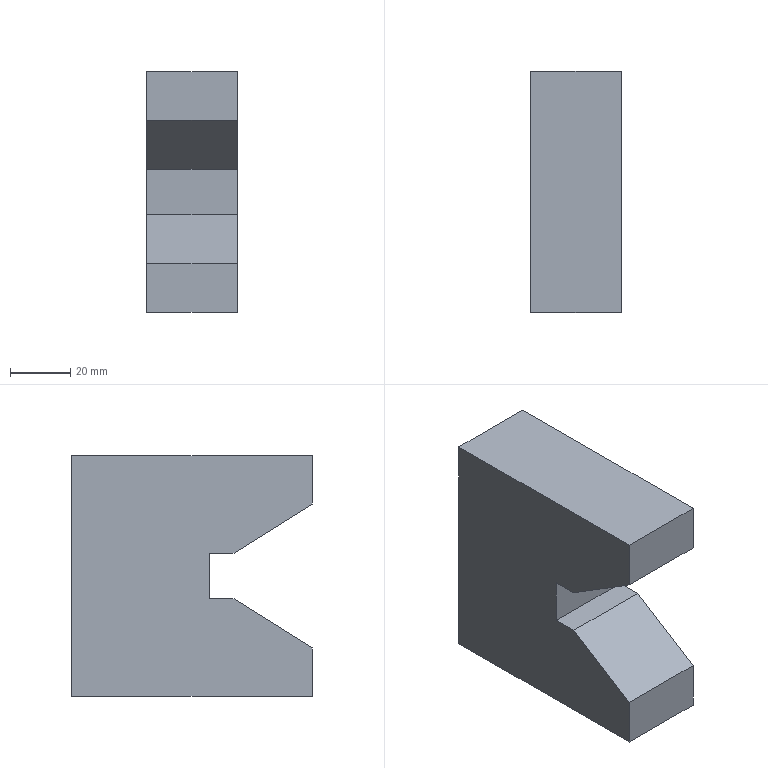Component | NX | MOVABLE_V_BLOCK | 1 solid | 14 faces | box 30 x 80 x 80 mm | volume 162754 mm3 | plane 13 | cylinder 1 | commonest cylinder face diameters 15 x1
STEP:
#1=CARTESIAN_POINT('',(0.,0.,0.));
#2=DIRECTION('',(0.,0.,1.));
#3=DIRECTION('',(1.,0.,0.));
#4=AXIS2_PLACEMENT_3D('',#1,#2,#3);
#5=CARTESIAN_POINT('',(39.511,118.604,6.098));
#6=VERTEX_POINT('',#5);
#7=CARTESIAN_POINT('',(39.511,144.658,22.378));
#8=VERTEX_POINT('',#7);
#9=CARTESIAN_POINT('',(39.511,118.604,6.098));
#10=DIRECTION('',(0.,0.848,0.5299));
#11=VECTOR('',#10,1.);
#12=LINE('',#9,#11);
#13=CARTESIAN_POINT('',(39.511,118.604,-10.));
#14=DIRECTION('',(-1.,0.,0.));
#15=DIRECTION('',(0.,-1.,0.));
#16=AXIS2_PLACEMENT_3D('',#13,#14,#15);
#17=PLANE('',#16);
#18=CARTESIAN_POINT('',(0.,16.098));
#19=DIRECTION('',(-0.848,0.5299));
#20=VECTOR('',#19,1.);
#21=LINE('',#18,#20);
#22=(GEOMETRIC_REPRESENTATION_CONTEXT(2)PARAMETRIC_REPRESENTATION_CONTEXT()REPRESENTATION_CONTEXT('',''));
#23=DEFINITIONAL_REPRESENTATION('',(#21),#22);
#24=PCURVE('',#17,#23);
#25=CARTESIAN_POINT('',(-280.489,118.604,6.098));
#26=DIRECTION('',(0.,0.5299,-0.848));
#27=DIRECTION('',(0.,-0.848,-0.5299));
#28=AXIS2_PLACEMENT_3D('',#25,#26,#27);
#29=PLANE('',#28);
#30=CARTESIAN_POINT('',(0.,-320.));
#31=DIRECTION('',(-1.,0.));
#32=VECTOR('',#31,1.);
#33=LINE('',#30,#32);
#34=(GEOMETRIC_REPRESENTATION_CONTEXT(2)PARAMETRIC_REPRESENTATION_CONTEXT()REPRESENTATION_CONTEXT('',''));
#35=DEFINITIONAL_REPRESENTATION('',(#33),#34);
#36=PCURVE('',#29,#35);
#37=SURFACE_CURVE('',#12,(#24,#36),.PCURVE_S1.);
#38=EDGE_CURVE('',#6,#8,#37,.T.);
#39=ORIENTED_EDGE('',*,*,#38,.F.);
#40=CARTESIAN_POINT('',(39.511,118.604,-10.));
#41=VERTEX_POINT('',#40);
#42=CARTESIAN_POINT('',(39.511,118.604,-10.));
#43=DIRECTION('',(0.,0.,1.));
#44=VECTOR('',#43,1.);
#45=LINE('',#42,#44);
#46=CARTESIAN_POINT('',(0.,0.));
#47=DIRECTION('',(0.,1.));
#48=VECTOR('',#47,1.);
#49=LINE('',#46,#48);
#50=(GEOMETRIC_REPRESENTATION_CONTEXT(2)PARAMETRIC_REPRESENTATION_CONTEXT()REPRESENTATION_CONTEXT('',''));
#51=DEFINITIONAL_REPRESENTATION('',(#49),#50);
#52=PCURVE('',#17,#51);
#53=CARTESIAN_POINT('',(39.511,118.604,-10.));
#54=DIRECTION('',(0.,-1.,0.));
#55=DIRECTION('',(0.,0.,1.));
#56=AXIS2_PLACEMENT_3D('',#53,#54,#55);
#57=PLANE('',#56);
#58=CARTESIAN_POINT('',(0.,0.));
#59=DIRECTION('',(1.,0.));
#60=VECTOR('',#59,1.);
#61=LINE('',#58,#60);
#62=(GEOMETRIC_REPRESENTATION_CONTEXT(2)PARAMETRIC_REPRESENTATION_CONTEXT()REPRESENTATION_CONTEXT('',''));
#63=DEFINITIONAL_REPRESENTATION('',(#61),#62);
#64=PCURVE('',#57,#63);
#65=SURFACE_CURVE('',#45,(#52,#64),.PCURVE_S1.);
#66=EDGE_CURVE('',#41,#6,#65,.T.);
#67=ORIENTED_EDGE('',*,*,#66,.F.);
#68=CARTESIAN_POINT('',(39.511,198.604,-10.));
#69=VERTEX_POINT('',#68);
#70=CARTESIAN_POINT('',(39.511,118.604,-10.));
#71=DIRECTION('',(0.,1.,0.));
#72=VECTOR('',#71,1.);
#73=LINE('',#70,#72);
#74=CARTESIAN_POINT('',(0.,0.));
#75=DIRECTION('',(-1.,0.));
#76=VECTOR('',#75,1.);
#77=LINE('',#74,#76);
#78=(GEOMETRIC_REPRESENTATION_CONTEXT(2)PARAMETRIC_REPRESENTATION_CONTEXT()REPRESENTATION_CONTEXT('',''));
#79=DEFINITIONAL_REPRESENTATION('',(#77),#78);
#80=PCURVE('',#17,#79);
#81=CARTESIAN_POINT('',(9.511,118.604,-10.));
#82=DIRECTION('',(0.,0.,1.));
#83=DIRECTION('',(-1.,0.,0.));
#84=AXIS2_PLACEMENT_3D('',#81,#82,#83);
#85=PLANE('',#84);
#86=CARTESIAN_POINT('',(-30.,0.));
#87=DIRECTION('',(0.,-1.));
#88=VECTOR('',#87,1.);
#89=LINE('',#86,#88);
#90=(GEOMETRIC_REPRESENTATION_CONTEXT(2)PARAMETRIC_REPRESENTATION_CONTEXT()REPRESENTATION_CONTEXT('',''));
#91=DEFINITIONAL_REPRESENTATION('',(#89),#90);
#92=PCURVE('',#85,#91);
#93=SURFACE_CURVE('',#73,(#80,#92),.PCURVE_S1.);
#94=EDGE_CURVE('',#41,#69,#93,.T.);
#95=ORIENTED_EDGE('',*,*,#94,.T.);
#96=CARTESIAN_POINT('',(39.511,198.604,70.));
#97=VERTEX_POINT('',#96);
#98=CARTESIAN_POINT('',(39.511,198.604,-10.));
#99=DIRECTION('',(0.,0.,1.));
#100=VECTOR('',#99,1.);
#101=LINE('',#98,#100);
#102=CARTESIAN_POINT('',(-80.,0.));
#103=DIRECTION('',(0.,1.));
#104=VECTOR('',#103,1.);
#105=LINE('',#102,#104);
#106=(GEOMETRIC_REPRESENTATION_CONTEXT(2)PARAMETRIC_REPRESENTATION_CONTEXT()REPRESENTATION_CONTEXT('',''));
#107=DEFINITIONAL_REPRESENTATION('',(#105),#106);
#108=PCURVE('',#17,#107);
#109=CARTESIAN_POINT('',(39.511,198.604,-10.));
#110=DIRECTION('',(0.,-1.,0.));
#111=DIRECTION('',(0.,0.,1.));
#112=AXIS2_PLACEMENT_3D('',#109,#110,#111);
#113=PLANE('',#112);
#114=CARTESIAN_POINT('',(0.,0.));
#115=DIRECTION('',(1.,0.));
#116=VECTOR('',#115,1.);
#117=LINE('',#114,#116);
#118=(GEOMETRIC_REPRESENTATION_CONTEXT(2)PARAMETRIC_REPRESENTATION_CONTEXT()REPRESENTATION_CONTEXT('',''));
#119=DEFINITIONAL_REPRESENTATION('',(#117),#118);
#120=PCURVE('',#113,#119);
#121=SURFACE_CURVE('',#101,(#108,#120),.PCURVE_S1.);
#122=EDGE_CURVE('',#69,#97,#121,.T.);
#123=ORIENTED_EDGE('',*,*,#122,.T.);
#124=CARTESIAN_POINT('',(39.511,118.604,70.));
#125=VERTEX_POINT('',#124);
#126=CARTESIAN_POINT('',(39.511,118.604,70.));
#127=DIRECTION('',(0.,1.,0.));
#128=VECTOR('',#127,1.);
#129=LINE('',#126,#128);
#130=CARTESIAN_POINT('',(0.,80.));
#131=DIRECTION('',(-1.,0.));
#132=VECTOR('',#131,1.);
#133=LINE('',#130,#132);
#134=(GEOMETRIC_REPRESENTATION_CONTEXT(2)PARAMETRIC_REPRESENTATION_CONTEXT()REPRESENTATION_CONTEXT('',''));
#135=DEFINITIONAL_REPRESENTATION('',(#133),#134);
#136=PCURVE('',#17,#135);
#137=CARTESIAN_POINT('',(39.511,118.604,70.));
#138=DIRECTION('',(0.,0.,-1.));
#139=DIRECTION('',(0.,-1.,0.));
#140=AXIS2_PLACEMENT_3D('',#137,#138,#139);
#141=PLANE('',#140);
#142=CARTESIAN_POINT('',(0.,0.));
#143=DIRECTION('',(-1.,0.));
#144=VECTOR('',#143,1.);
#145=LINE('',#142,#144);
#146=(GEOMETRIC_REPRESENTATION_CONTEXT(2)PARAMETRIC_REPRESENTATION_CONTEXT()REPRESENTATION_CONTEXT('',''));
#147=DEFINITIONAL_REPRESENTATION('',(#145),#146);
#148=PCURVE('',#141,#147);
#149=SURFACE_CURVE('',#129,(#136,#148),.PCURVE_S1.);
#150=EDGE_CURVE('',#125,#97,#149,.T.);
#151=ORIENTED_EDGE('',*,*,#150,.F.);
#152=CARTESIAN_POINT('',(39.511,118.604,53.902));
#153=VERTEX_POINT('',#152);
#154=CARTESIAN_POINT('',(39.511,118.604,-10.));
#155=DIRECTION('',(0.,0.,1.));
#156=VECTOR('',#155,1.);
#157=LINE('',#154,#156);
#158=CARTESIAN_POINT('',(0.,0.));
#159=DIRECTION('',(0.,1.));
#160=VECTOR('',#159,1.);
#161=LINE('',#158,#160);
#162=(GEOMETRIC_REPRESENTATION_CONTEXT(2)PARAMETRIC_REPRESENTATION_CONTEXT()REPRESENTATION_CONTEXT('',''));
#163=DEFINITIONAL_REPRESENTATION('',(#161),#162);
#164=PCURVE('',#17,#163);
#165=CARTESIAN_POINT('',(39.511,118.604,-10.));
#166=DIRECTION('',(0.,-1.,0.));
#167=DIRECTION('',(0.,0.,1.));
#168=AXIS2_PLACEMENT_3D('',#165,#166,#167);
#169=PLANE('',#168);
#170=CARTESIAN_POINT('',(0.,0.));
#171=DIRECTION('',(1.,0.));
#172=VECTOR('',#171,1.);
#173=LINE('',#170,#172);
#174=(GEOMETRIC_REPRESENTATION_CONTEXT(2)PARAMETRIC_REPRESENTATION_CONTEXT()REPRESENTATION_CONTEXT('',''));
#175=DEFINITIONAL_REPRESENTATION('',(#173),#174);
#176=PCURVE('',#169,#175);
#177=SURFACE_CURVE('',#157,(#164,#176),.PCURVE_S1.);
#178=EDGE_CURVE('',#153,#125,#177,.T.);
#179=ORIENTED_EDGE('',*,*,#178,.F.);
#180=CARTESIAN_POINT('',(39.511,144.658,37.622));
#181=VERTEX_POINT('',#180);
#182=CARTESIAN_POINT('',(39.511,144.658,37.622));
#183=DIRECTION('',(0.,-0.848,0.5299));
#184=VECTOR('',#183,1.);
#185=LINE('',#182,#184);
#186=CARTESIAN_POINT('',(-26.054,47.622));
#187=DIRECTION('',(0.848,0.5299));
#188=VECTOR('',#187,1.);
#189=LINE('',#186,#188);
#190=(GEOMETRIC_REPRESENTATION_CONTEXT(2)PARAMETRIC_REPRESENTATION_CONTEXT()REPRESENTATION_CONTEXT('',''));
#191=DEFINITIONAL_REPRESENTATION('',(#189),#190);
#192=PCURVE('',#17,#191);
#193=CARTESIAN_POINT('',(-280.489,144.658,37.622));
#194=DIRECTION('',(0.,0.5299,0.848));
#195=DIRECTION('',(0.,0.848,-0.5299));
#196=AXIS2_PLACEMENT_3D('',#193,#194,#195);
#197=PLANE('',#196);
#198=CARTESIAN_POINT('',(0.,-320.));
#199=DIRECTION('',(-1.,0.));
#200=VECTOR('',#199,1.);
#201=LINE('',#198,#200);
#202=(GEOMETRIC_REPRESENTATION_CONTEXT(2)PARAMETRIC_REPRESENTATION_CONTEXT()REPRESENTATION_CONTEXT('',''));
#203=DEFINITIONAL_REPRESENTATION('',(#201),#202);
#204=PCURVE('',#197,#203);
#205=SURFACE_CURVE('',#185,(#192,#204),.PCURVE_S1.);
#206=EDGE_CURVE('',#181,#153,#205,.T.);
#207=ORIENTED_EDGE('',*,*,#206,.F.);
#208=CARTESIAN_POINT('',(39.511,152.798,37.622));
#209=VERTEX_POINT('',#208);
#210=CARTESIAN_POINT('',(39.511,152.798,37.622));
#211=DIRECTION('',(0.,-1.,0.));
#212=VECTOR('',#211,1.);
#213=LINE('',#210,#212);
#214=CARTESIAN_POINT('',(-34.194,47.622));
#215=DIRECTION('',(1.,0.));
#216=VECTOR('',#215,1.);
#217=LINE('',#214,#216);
#218=(GEOMETRIC_REPRESENTATION_CONTEXT(2)PARAMETRIC_REPRESENTATION_CONTEXT()REPRESENTATION_CONTEXT('',''));
#219=DEFINITIONAL_REPRESENTATION('',(#217),#218);
#220=PCURVE('',#17,#219);
#221=CARTESIAN_POINT('',(-280.489,152.798,37.622));
#222=DIRECTION('',(0.,0.,1.));
#223=DIRECTION('',(0.,1.,0.));
#224=AXIS2_PLACEMENT_3D('',#221,#222,#223);
#225=PLANE('',#224);
#226=CARTESIAN_POINT('',(0.,-320.));
#227=DIRECTION('',(-1.,0.));
#228=VECTOR('',#227,1.);
#229=LINE('',#226,#228);
#230=(GEOMETRIC_REPRESENTATION_CONTEXT(2)PARAMETRIC_REPRESENTATION_CONTEXT()REPRESENTATION_CONTEXT('',''));
#231=DEFINITIONAL_REPRESENTATION('',(#229),#230);
#232=PCURVE('',#225,#231);
#233=SURFACE_CURVE('',#213,(#220,#232),.PCURVE_S1.);
#234=EDGE_CURVE('',#209,#181,#233,.T.);
#235=ORIENTED_EDGE('',*,*,#234,.F.);
#236=CARTESIAN_POINT('',(39.511,152.798,22.378));
#237=VERTEX_POINT('',#236);
#238=CARTESIAN_POINT('',(39.511,152.798,22.378));
#239=DIRECTION('',(0.,0.,1.));
#240=VECTOR('',#239,1.);
#241=LINE('',#238,#240);
#242=CARTESIAN_POINT('',(-34.194,32.378));
#243=DIRECTION('',(0.,1.));
#244=VECTOR('',#243,1.);
#245=LINE('',#242,#244);
#246=(GEOMETRIC_REPRESENTATION_CONTEXT(2)PARAMETRIC_REPRESENTATION_CONTEXT()REPRESENTATION_CONTEXT('',''));
#247=DEFINITIONAL_REPRESENTATION('',(#245),#246);
#248=PCURVE('',#17,#247);
#249=CARTESIAN_POINT('',(-280.489,152.798,22.378));
#250=DIRECTION('',(0.,1.,0.));
#251=DIRECTION('',(0.,0.,-1.));
#252=AXIS2_PLACEMENT_3D('',#249,#250,#251);
#253=PLANE('',#252);
#254=CARTESIAN_POINT('',(0.,-320.));
#255=DIRECTION('',(-1.,0.));
#256=VECTOR('',#255,1.);
#257=LINE('',#254,#256);
#258=(GEOMETRIC_REPRESENTATION_CONTEXT(2)PARAMETRIC_REPRESENTATION_CONTEXT()REPRESENTATION_CONTEXT('',''));
#259=DEFINITIONAL_REPRESENTATION('',(#257),#258);
#260=PCURVE('',#253,#259);
#261=SURFACE_CURVE('',#241,(#248,#260),.PCURVE_S1.);
#262=EDGE_CURVE('',#237,#209,#261,.T.);
#263=ORIENTED_EDGE('',*,*,#262,.F.);
#264=CARTESIAN_POINT('',(39.511,144.658,22.378));
#265=DIRECTION('',(0.,1.,0.));
#266=VECTOR('',#265,1.);
#267=LINE('',#264,#266);
#268=CARTESIAN_POINT('',(-26.054,32.378));
#269=DIRECTION('',(-1.,0.));
#270=VECTOR('',#269,1.);
#271=LINE('',#268,#270);
#272=(GEOMETRIC_REPRESENTATION_CONTEXT(2)PARAMETRIC_REPRESENTATION_CONTEXT()REPRESENTATION_CONTEXT('',''));
#273=DEFINITIONAL_REPRESENTATION('',(#271),#272);
#274=PCURVE('',#17,#273);
#275=CARTESIAN_POINT('',(-280.489,144.658,22.378));
#276=DIRECTION('',(0.,0.,-1.));
#277=DIRECTION('',(0.,-1.,0.));
#278=AXIS2_PLACEMENT_3D('',#275,#276,#277);
#279=PLANE('',#278);
#280=CARTESIAN_POINT('',(0.,-320.));
#281=DIRECTION('',(-1.,0.));
#282=VECTOR('',#281,1.);
#283=LINE('',#280,#282);
#284=(GEOMETRIC_REPRESENTATION_CONTEXT(2)PARAMETRIC_REPRESENTATION_CONTEXT()REPRESENTATION_CONTEXT('',''));
#285=DEFINITIONAL_REPRESENTATION('',(#283),#284);
#286=PCURVE('',#279,#285);
#287=SURFACE_CURVE('',#267,(#274,#286),.PCURVE_S1.);
#288=EDGE_CURVE('',#8,#237,#287,.T.);
#289=ORIENTED_EDGE('',*,*,#288,.F.);
#290=EDGE_LOOP('',(#39,#67,#95,#123,#151,#179,#207,#235,#263,#289));
#291=FACE_BOUND('',#290,.T.);
#292=ADVANCED_FACE('',(#291),#17,.F.);
#293=CARTESIAN_POINT('',(9.511,118.604,70.));
#294=VERTEX_POINT('',#293);
#295=CARTESIAN_POINT('',(9.511,118.604,53.902));
#296=VERTEX_POINT('',#295);
#297=CARTESIAN_POINT('',(9.511,118.604,70.));
#298=DIRECTION('',(0.,0.,-1.));
#299=VECTOR('',#298,1.);
#300=LINE('',#297,#299);
#301=CARTESIAN_POINT('',(80.,30.));
#302=DIRECTION('',(-1.,-0.));
#303=VECTOR('',#302,1.);
#304=LINE('',#301,#303);
#305=(GEOMETRIC_REPRESENTATION_CONTEXT(2)PARAMETRIC_REPRESENTATION_CONTEXT()REPRESENTATION_CONTEXT('',''));
#306=DEFINITIONAL_REPRESENTATION('',(#304),#305);
#307=PCURVE('',#169,#306);
#308=CARTESIAN_POINT('',(9.511,118.604,70.));
#309=DIRECTION('',(1.,0.,0.));
#310=DIRECTION('',(-0.,0.,1.));
#311=AXIS2_PLACEMENT_3D('',#308,#309,#310);
#312=PLANE('',#311);
#313=CARTESIAN_POINT('',(0.,0.));
#314=DIRECTION('',(-1.,0.));
#315=VECTOR('',#314,1.);
#316=LINE('',#313,#315);
#317=(GEOMETRIC_REPRESENTATION_CONTEXT(2)PARAMETRIC_REPRESENTATION_CONTEXT()REPRESENTATION_CONTEXT('',''));
#318=DEFINITIONAL_REPRESENTATION('',(#316),#317);
#319=PCURVE('',#312,#318);
#320=SURFACE_CURVE('',#300,(#307,#319),.PCURVE_S1.);
#321=EDGE_CURVE('',#294,#296,#320,.T.);
#322=ORIENTED_EDGE('',*,*,#321,.T.);
#323=CARTESIAN_POINT('',(-280.489,118.604,53.902));
#324=DIRECTION('',(1.,0.,0.));
#325=VECTOR('',#324,1.);
#326=LINE('',#323,#325);
#327=CARTESIAN_POINT('',(63.902,320.));
#328=DIRECTION('',(0.,-1.));
#329=VECTOR('',#328,1.);
#330=LINE('',#327,#329);
#331=(GEOMETRIC_REPRESENTATION_CONTEXT(2)PARAMETRIC_REPRESENTATION_CONTEXT()REPRESENTATION_CONTEXT('',''));
#332=DEFINITIONAL_REPRESENTATION('',(#330),#331);
#333=PCURVE('',#169,#332);
#334=CARTESIAN_POINT('',(-30.722,0.));
#335=DIRECTION('',(0.,-1.));
#336=VECTOR('',#335,1.);
#337=LINE('',#334,#336);
#338=(GEOMETRIC_REPRESENTATION_CONTEXT(2)PARAMETRIC_REPRESENTATION_CONTEXT()REPRESENTATION_CONTEXT('',''));
#339=DEFINITIONAL_REPRESENTATION('',(#337),#338);
#340=PCURVE('',#197,#339);
#341=SURFACE_CURVE('',#326,(#333,#340),.PCURVE_S1.);
#342=EDGE_CURVE('',#296,#153,#341,.T.);
#343=ORIENTED_EDGE('',*,*,#342,.T.);
#344=ORIENTED_EDGE('',*,*,#178,.T.);
#345=CARTESIAN_POINT('',(39.511,118.604,70.));
#346=DIRECTION('',(-1.,0.,0.));
#347=VECTOR('',#346,1.);
#348=LINE('',#345,#347);
#349=CARTESIAN_POINT('',(80.,0.));
#350=DIRECTION('',(0.,1.));
#351=VECTOR('',#350,1.);
#352=LINE('',#349,#351);
#353=(GEOMETRIC_REPRESENTATION_CONTEXT(2)PARAMETRIC_REPRESENTATION_CONTEXT()REPRESENTATION_CONTEXT('',''));
#354=DEFINITIONAL_REPRESENTATION('',(#352),#353);
#355=PCURVE('',#169,#354);
#356=CARTESIAN_POINT('',(0.,0.));
#357=DIRECTION('',(0.,1.));
#358=VECTOR('',#357,1.);
#359=LINE('',#356,#358);
#360=(GEOMETRIC_REPRESENTATION_CONTEXT(2)PARAMETRIC_REPRESENTATION_CONTEXT()REPRESENTATION_CONTEXT('',''));
#361=DEFINITIONAL_REPRESENTATION('',(#359),#360);
#362=PCURVE('',#141,#361);
#363=SURFACE_CURVE('',#348,(#355,#362),.PCURVE_S1.);
#364=EDGE_CURVE('',#125,#294,#363,.T.);
#365=ORIENTED_EDGE('',*,*,#364,.T.);
#366=EDGE_LOOP('',(#322,#343,#344,#365));
#367=FACE_BOUND('',#366,.T.);
#368=ADVANCED_FACE('',(#367),#169,.T.);
#369=CARTESIAN_POINT('',(9.511,198.604,-10.));
#370=VERTEX_POINT('',#369);
#371=CARTESIAN_POINT('',(9.511,198.604,-10.));
#372=DIRECTION('',(1.,0.,-0.));
#373=VECTOR('',#372,1.);
#374=LINE('',#371,#373);
#375=CARTESIAN_POINT('',(0.,-80.));
#376=DIRECTION('',(-1.,0.));
#377=VECTOR('',#376,1.);
#378=LINE('',#375,#377);
#379=(GEOMETRIC_REPRESENTATION_CONTEXT(2)PARAMETRIC_REPRESENTATION_CONTEXT()REPRESENTATION_CONTEXT('',''));
#380=DEFINITIONAL_REPRESENTATION('',(#378),#379);
#381=PCURVE('',#85,#380);
#382=CARTESIAN_POINT('',(0.,30.));
#383=DIRECTION('',(-0.,-1.));
#384=VECTOR('',#383,1.);
#385=LINE('',#382,#384);
#386=(GEOMETRIC_REPRESENTATION_CONTEXT(2)PARAMETRIC_REPRESENTATION_CONTEXT()REPRESENTATION_CONTEXT('',''));
#387=DEFINITIONAL_REPRESENTATION('',(#385),#386);
#388=PCURVE('',#113,#387);
#389=SURFACE_CURVE('',#374,(#381,#388),.PCURVE_S1.);
#390=EDGE_CURVE('',#370,#69,#389,.T.);
#391=ORIENTED_EDGE('',*,*,#390,.T.);
#392=ORIENTED_EDGE('',*,*,#94,.F.);
#393=CARTESIAN_POINT('',(9.511,118.604,-10.));
#394=VERTEX_POINT('',#393);
#395=CARTESIAN_POINT('',(9.511,118.604,-10.));
#396=DIRECTION('',(1.,0.,-0.));
#397=VECTOR('',#396,1.);
#398=LINE('',#395,#397);
#399=CARTESIAN_POINT('',(0.,0.));
#400=DIRECTION('',(-1.,0.));
#401=VECTOR('',#400,1.);
#402=LINE('',#399,#401);
#403=(GEOMETRIC_REPRESENTATION_CONTEXT(2)PARAMETRIC_REPRESENTATION_CONTEXT()REPRESENTATION_CONTEXT('',''));
#404=DEFINITIONAL_REPRESENTATION('',(#402),#403);
#405=PCURVE('',#85,#404);
#406=CARTESIAN_POINT('',(0.,30.));
#407=DIRECTION('',(-0.,-1.));
#408=VECTOR('',#407,1.);
#409=LINE('',#406,#408);
#410=(GEOMETRIC_REPRESENTATION_CONTEXT(2)PARAMETRIC_REPRESENTATION_CONTEXT()REPRESENTATION_CONTEXT('',''));
#411=DEFINITIONAL_REPRESENTATION('',(#409),#410);
#412=PCURVE('',#57,#411);
#413=SURFACE_CURVE('',#398,(#405,#412),.PCURVE_S1.);
#414=EDGE_CURVE('',#394,#41,#413,.T.);
#415=ORIENTED_EDGE('',*,*,#414,.F.);
#416=CARTESIAN_POINT('',(9.511,118.604,-10.));
#417=DIRECTION('',(0.,1.,0.));
#418=VECTOR('',#417,1.);
#419=LINE('',#416,#418);
#420=CARTESIAN_POINT('',(0.,0.));
#421=DIRECTION('',(0.,-1.));
#422=VECTOR('',#421,1.);
#423=LINE('',#420,#422);
#424=(GEOMETRIC_REPRESENTATION_CONTEXT(2)PARAMETRIC_REPRESENTATION_CONTEXT()REPRESENTATION_CONTEXT('',''));
#425=DEFINITIONAL_REPRESENTATION('',(#423),#424);
#426=PCURVE('',#85,#425);
#427=CARTESIAN_POINT('',(-80.,0.));
#428=DIRECTION('',(0.,-1.));
#429=VECTOR('',#428,1.);
#430=LINE('',#427,#429);
#431=(GEOMETRIC_REPRESENTATION_CONTEXT(2)PARAMETRIC_REPRESENTATION_CONTEXT()REPRESENTATION_CONTEXT('',''));
#432=DEFINITIONAL_REPRESENTATION('',(#430),#431);
#433=PCURVE('',#312,#432);
#434=SURFACE_CURVE('',#419,(#426,#433),.PCURVE_S1.);
#435=EDGE_CURVE('',#394,#370,#434,.T.);
#436=ORIENTED_EDGE('',*,*,#435,.T.);
#437=EDGE_LOOP('',(#391,#392,#415,#436));
#438=FACE_BOUND('',#437,.T.);
#439=ADVANCED_FACE('',(#438),#85,.F.);
#440=CARTESIAN_POINT('',(9.511,198.604,70.));
#441=VERTEX_POINT('',#440);
#442=CARTESIAN_POINT('',(39.511,198.604,70.));
#443=DIRECTION('',(-1.,0.,0.));
#444=VECTOR('',#443,1.);
#445=LINE('',#442,#444);
#446=CARTESIAN_POINT('',(-80.,0.));
#447=DIRECTION('',(0.,1.));
#448=VECTOR('',#447,1.);
#449=LINE('',#446,#448);
#450=(GEOMETRIC_REPRESENTATION_CONTEXT(2)PARAMETRIC_REPRESENTATION_CONTEXT()REPRESENTATION_CONTEXT('',''));
#451=DEFINITIONAL_REPRESENTATION('',(#449),#450);
#452=PCURVE('',#141,#451);
#453=CARTESIAN_POINT('',(80.,0.));
#454=DIRECTION('',(0.,1.));
#455=VECTOR('',#454,1.);
#456=LINE('',#453,#455);
#457=(GEOMETRIC_REPRESENTATION_CONTEXT(2)PARAMETRIC_REPRESENTATION_CONTEXT()REPRESENTATION_CONTEXT('',''));
#458=DEFINITIONAL_REPRESENTATION('',(#456),#457);
#459=PCURVE('',#113,#458);
#460=SURFACE_CURVE('',#445,(#452,#459),.PCURVE_S1.);
#461=EDGE_CURVE('',#97,#441,#460,.T.);
#462=ORIENTED_EDGE('',*,*,#461,.T.);
#463=CARTESIAN_POINT('',(9.511,118.604,70.));
#464=DIRECTION('',(0.,1.,0.));
#465=VECTOR('',#464,1.);
#466=LINE('',#463,#465);
#467=CARTESIAN_POINT('',(0.,30.));
#468=DIRECTION('',(-1.,0.));
#469=VECTOR('',#468,1.);
#470=LINE('',#467,#469);
#471=(GEOMETRIC_REPRESENTATION_CONTEXT(2)PARAMETRIC_REPRESENTATION_CONTEXT()REPRESENTATION_CONTEXT('',''));
#472=DEFINITIONAL_REPRESENTATION('',(#470),#471);
#473=PCURVE('',#141,#472);
#474=CARTESIAN_POINT('',(0.,0.));
#475=DIRECTION('',(0.,-1.));
#476=VECTOR('',#475,1.);
#477=LINE('',#474,#476);
#478=(GEOMETRIC_REPRESENTATION_CONTEXT(2)PARAMETRIC_REPRESENTATION_CONTEXT()REPRESENTATION_CONTEXT('',''));
#479=DEFINITIONAL_REPRESENTATION('',(#477),#478);
#480=PCURVE('',#312,#479);
#481=SURFACE_CURVE('',#466,(#473,#480),.PCURVE_S1.);
#482=EDGE_CURVE('',#294,#441,#481,.T.);
#483=ORIENTED_EDGE('',*,*,#482,.F.);
#484=ORIENTED_EDGE('',*,*,#364,.F.);
#485=ORIENTED_EDGE('',*,*,#150,.T.);
#486=EDGE_LOOP('',(#462,#483,#484,#485));
#487=FACE_BOUND('',#486,.T.);
#488=ADVANCED_FACE('',(#487),#141,.F.);
#489=CARTESIAN_POINT('',(9.511,118.604,6.098));
#490=VERTEX_POINT('',#489);
#491=CARTESIAN_POINT('',(9.511,118.604,70.));
#492=DIRECTION('',(0.,0.,-1.));
#493=VECTOR('',#492,1.);
#494=LINE('',#491,#493);
#495=CARTESIAN_POINT('',(0.,0.));
#496=DIRECTION('',(-1.,0.));
#497=VECTOR('',#496,1.);
#498=LINE('',#495,#497);
#499=(GEOMETRIC_REPRESENTATION_CONTEXT(2)PARAMETRIC_REPRESENTATION_CONTEXT()REPRESENTATION_CONTEXT('',''));
#500=DEFINITIONAL_REPRESENTATION('',(#498),#499);
#501=PCURVE('',#312,#500);
#502=CARTESIAN_POINT('',(80.,30.));
#503=DIRECTION('',(-1.,-0.));
#504=VECTOR('',#503,1.);
#505=LINE('',#502,#504);
#506=(GEOMETRIC_REPRESENTATION_CONTEXT(2)PARAMETRIC_REPRESENTATION_CONTEXT()REPRESENTATION_CONTEXT('',''));
#507=DEFINITIONAL_REPRESENTATION('',(#505),#506);
#508=PCURVE('',#57,#507);
#509=SURFACE_CURVE('',#494,(#501,#508),.PCURVE_S1.);
#510=EDGE_CURVE('',#490,#394,#509,.T.);
#511=ORIENTED_EDGE('',*,*,#510,.F.);
#512=CARTESIAN_POINT('',(9.511,144.658,22.378));
#513=VERTEX_POINT('',#512);
#514=CARTESIAN_POINT('',(9.511,147.321,24.042));
#515=DIRECTION('',(-0.,0.848,0.5299));
#516=VECTOR('',#515,1.);
#517=LINE('',#514,#516);
#518=CARTESIAN_POINT('',(-45.958,-28.718));
#519=DIRECTION('',(0.5299,-0.848));
#520=VECTOR('',#519,1.);
#521=LINE('',#518,#520);
#522=(GEOMETRIC_REPRESENTATION_CONTEXT(2)PARAMETRIC_REPRESENTATION_CONTEXT()REPRESENTATION_CONTEXT('',''));
#523=DEFINITIONAL_REPRESENTATION('',(#521),#522);
#524=PCURVE('',#312,#523);
#525=CARTESIAN_POINT('',(-33.863,-290.));
#526=DIRECTION('',(-1.,0.));
#527=VECTOR('',#526,1.);
#528=LINE('',#525,#527);
#529=(GEOMETRIC_REPRESENTATION_CONTEXT(2)PARAMETRIC_REPRESENTATION_CONTEXT()REPRESENTATION_CONTEXT('',''));
#530=DEFINITIONAL_REPRESENTATION('',(#528),#529);
#531=PCURVE('',#29,#530);
#532=SURFACE_CURVE('',#517,(#524,#531),.PCURVE_S1.);
#533=EDGE_CURVE('',#490,#513,#532,.T.);
#534=ORIENTED_EDGE('',*,*,#533,.T.);
#535=CARTESIAN_POINT('',(9.511,152.798,22.378));
#536=VERTEX_POINT('',#535);
#537=CARTESIAN_POINT('',(9.511,118.604,22.378));
#538=DIRECTION('',(0.,1.,0.));
#539=VECTOR('',#538,1.);
#540=LINE('',#537,#539);
#541=CARTESIAN_POINT('',(-47.622,0.));
#542=DIRECTION('',(0.,-1.));
#543=VECTOR('',#542,1.);
#544=LINE('',#541,#543);
#545=(GEOMETRIC_REPRESENTATION_CONTEXT(2)PARAMETRIC_REPRESENTATION_CONTEXT()REPRESENTATION_CONTEXT('',''));
#546=DEFINITIONAL_REPRESENTATION('',(#544),#545);
#547=PCURVE('',#312,#546);
#548=CARTESIAN_POINT('',(26.054,-290.));
#549=DIRECTION('',(-1.,0.));
#550=VECTOR('',#549,1.);
#551=LINE('',#548,#550);
#552=(GEOMETRIC_REPRESENTATION_CONTEXT(2)PARAMETRIC_REPRESENTATION_CONTEXT()REPRESENTATION_CONTEXT('',''));
#553=DEFINITIONAL_REPRESENTATION('',(#551),#552);
#554=PCURVE('',#279,#553);
#555=SURFACE_CURVE('',#540,(#547,#554),.PCURVE_S1.);
#556=EDGE_CURVE('',#513,#536,#555,.T.);
#557=ORIENTED_EDGE('',*,*,#556,.T.);
#558=CARTESIAN_POINT('',(9.511,152.798,37.622));
#559=VERTEX_POINT('',#558);
#560=CARTESIAN_POINT('',(9.511,152.798,70.));
#561=DIRECTION('',(-0.,0.,1.));
#562=VECTOR('',#561,1.);
#563=LINE('',#560,#562);
#564=CARTESIAN_POINT('',(0.,-34.194));
#565=DIRECTION('',(1.,0.));
#566=VECTOR('',#565,1.);
#567=LINE('',#564,#566);
#568=(GEOMETRIC_REPRESENTATION_CONTEXT(2)PARAMETRIC_REPRESENTATION_CONTEXT()REPRESENTATION_CONTEXT('',''));
#569=DEFINITIONAL_REPRESENTATION('',(#567),#568);
#570=PCURVE('',#312,#569);
#571=CARTESIAN_POINT('',(-47.622,-290.));
#572=DIRECTION('',(-1.,0.));
#573=VECTOR('',#572,1.);
#574=LINE('',#571,#573);
#575=(GEOMETRIC_REPRESENTATION_CONTEXT(2)PARAMETRIC_REPRESENTATION_CONTEXT()REPRESENTATION_CONTEXT('',''));
#576=DEFINITIONAL_REPRESENTATION('',(#574),#575);
#577=PCURVE('',#253,#576);
#578=SURFACE_CURVE('',#563,(#570,#577),.PCURVE_S1.);
#579=EDGE_CURVE('',#536,#559,#578,.T.);
#580=ORIENTED_EDGE('',*,*,#579,.T.);
#581=CARTESIAN_POINT('',(9.511,144.658,37.622));
#582=VERTEX_POINT('',#581);
#583=CARTESIAN_POINT('',(9.511,118.604,37.622));
#584=DIRECTION('',(0.,-1.,0.));
#585=VECTOR('',#584,1.);
#586=LINE('',#583,#585);
#587=CARTESIAN_POINT('',(-32.378,0.));
#588=DIRECTION('',(0.,1.));
#589=VECTOR('',#588,1.);
#590=LINE('',#587,#589);
#591=(GEOMETRIC_REPRESENTATION_CONTEXT(2)PARAMETRIC_REPRESENTATION_CONTEXT()REPRESENTATION_CONTEXT('',''));
#592=DEFINITIONAL_REPRESENTATION('',(#590),#591);
#593=PCURVE('',#312,#592);
#594=CARTESIAN_POINT('',(-34.194,-290.));
#595=DIRECTION('',(-1.,0.));
#596=VECTOR('',#595,1.);
#597=LINE('',#594,#596);
#598=(GEOMETRIC_REPRESENTATION_CONTEXT(2)PARAMETRIC_REPRESENTATION_CONTEXT()REPRESENTATION_CONTEXT('',''));
#599=DEFINITIONAL_REPRESENTATION('',(#597),#598);
#600=PCURVE('',#225,#599);
#601=SURFACE_CURVE('',#586,(#593,#600),.PCURVE_S1.);
#602=EDGE_CURVE('',#559,#582,#601,.T.);
#603=ORIENTED_EDGE('',*,*,#602,.T.);
#604=CARTESIAN_POINT('',(9.511,111.37,58.423));
#605=DIRECTION('',(-0.,-0.848,0.5299));
#606=VECTOR('',#605,1.);
#607=LINE('',#604,#606);
#608=CARTESIAN_POINT('',(-11.577,7.234));
#609=DIRECTION('',(0.5299,0.848));
#610=VECTOR('',#609,1.);
#611=LINE('',#608,#610);
#612=(GEOMETRIC_REPRESENTATION_CONTEXT(2)PARAMETRIC_REPRESENTATION_CONTEXT()REPRESENTATION_CONTEXT('',''));
#613=DEFINITIONAL_REPRESENTATION('',(#611),#612);
#614=PCURVE('',#312,#613);
#615=CARTESIAN_POINT('',(-39.253,-290.));
#616=DIRECTION('',(-1.,0.));
#617=VECTOR('',#616,1.);
#618=LINE('',#615,#617);
#619=(GEOMETRIC_REPRESENTATION_CONTEXT(2)PARAMETRIC_REPRESENTATION_CONTEXT()REPRESENTATION_CONTEXT('',''));
#620=DEFINITIONAL_REPRESENTATION('',(#618),#619);
#621=PCURVE('',#197,#620);
#622=SURFACE_CURVE('',#607,(#614,#621),.PCURVE_S1.);
#623=EDGE_CURVE('',#582,#296,#622,.T.);
#624=ORIENTED_EDGE('',*,*,#623,.T.);
#625=ORIENTED_EDGE('',*,*,#321,.F.);
#626=ORIENTED_EDGE('',*,*,#482,.T.);
#627=CARTESIAN_POINT('',(9.511,198.604,70.));
#628=DIRECTION('',(0.,0.,-1.));
#629=VECTOR('',#628,1.);
#630=LINE('',#627,#629);
#631=CARTESIAN_POINT('',(0.,-80.));
#632=DIRECTION('',(-1.,0.));
#633=VECTOR('',#632,1.);
#634=LINE('',#631,#633);
#635=(GEOMETRIC_REPRESENTATION_CONTEXT(2)PARAMETRIC_REPRESENTATION_CONTEXT()REPRESENTATION_CONTEXT('',''));
#636=DEFINITIONAL_REPRESENTATION('',(#634),#635);
#637=PCURVE('',#312,#636);
#638=CARTESIAN_POINT('',(80.,30.));
#639=DIRECTION('',(-1.,-0.));
#640=VECTOR('',#639,1.);
#641=LINE('',#638,#640);
#642=(GEOMETRIC_REPRESENTATION_CONTEXT(2)PARAMETRIC_REPRESENTATION_CONTEXT()REPRESENTATION_CONTEXT('',''));
#643=DEFINITIONAL_REPRESENTATION('',(#641),#642);
#644=PCURVE('',#113,#643);
#645=SURFACE_CURVE('',#630,(#637,#644),.PCURVE_S1.);
#646=EDGE_CURVE('',#441,#370,#645,.T.);
#647=ORIENTED_EDGE('',*,*,#646,.T.);
#648=ORIENTED_EDGE('',*,*,#435,.F.);
#649=EDGE_LOOP('',(#511,#534,#557,#580,#603,#624,#625,#626,#647,#648));
#650=FACE_BOUND('',#649,.T.);
#651=ADVANCED_FACE('',(#650),#312,.F.);
#652=CARTESIAN_POINT('',(-280.489,118.604,6.098));
#653=DIRECTION('',(1.,0.,0.));
#654=VECTOR('',#653,1.);
#655=LINE('',#652,#654);
#656=CARTESIAN_POINT('',(16.098,320.));
#657=DIRECTION('',(0.,-1.));
#658=VECTOR('',#657,1.);
#659=LINE('',#656,#658);
#660=(GEOMETRIC_REPRESENTATION_CONTEXT(2)PARAMETRIC_REPRESENTATION_CONTEXT()REPRESENTATION_CONTEXT('',''));
#661=DEFINITIONAL_REPRESENTATION('',(#659),#660);
#662=PCURVE('',#57,#661);
#663=CARTESIAN_POINT('',(0.,0.));
#664=DIRECTION('',(0.,-1.));
#665=VECTOR('',#664,1.);
#666=LINE('',#663,#665);
#667=(GEOMETRIC_REPRESENTATION_CONTEXT(2)PARAMETRIC_REPRESENTATION_CONTEXT()REPRESENTATION_CONTEXT('',''));
#668=DEFINITIONAL_REPRESENTATION('',(#666),#667);
#669=PCURVE('',#29,#668);
#670=SURFACE_CURVE('',#655,(#662,#669),.PCURVE_S1.);
#671=EDGE_CURVE('',#490,#6,#670,.T.);
#672=ORIENTED_EDGE('',*,*,#671,.F.);
#673=ORIENTED_EDGE('',*,*,#510,.T.);
#674=ORIENTED_EDGE('',*,*,#414,.T.);
#675=ORIENTED_EDGE('',*,*,#66,.T.);
#676=EDGE_LOOP('',(#672,#673,#674,#675));
#677=FACE_BOUND('',#676,.T.);
#678=ADVANCED_FACE('',(#677),#57,.T.);
#679=CARTESIAN_POINT('',(24.511,198.604,37.5));
#680=VERTEX_POINT('',#679);
#681=CARTESIAN_POINT('',(24.511,198.604,30.));
#682=DIRECTION('',(0.,1.,0.));
#683=DIRECTION('',(0.,0.,1.));
#684=AXIS2_PLACEMENT_3D('',#681,#682,#683);
#685=CIRCLE('',#684,7.5);
#686=CARTESIAN_POINT('',(47.5,15.));
#687=CARTESIAN_POINT('',(47.5,2.01));
#688=CARTESIAN_POINT('',(36.25,8.505));
#689=CARTESIAN_POINT('',(25.,15.));
#690=CARTESIAN_POINT('',(36.25,21.495));
#691=CARTESIAN_POINT('',(47.5,27.99));
#692=CARTESIAN_POINT('',(47.5,15.));
#693=(BOUNDED_CURVE()B_SPLINE_CURVE(2,(#686,#687,#688,#689,#690,#691,#692),.UNSPECIFIED.,.T.,.F.)B_SPLINE_CURVE_WITH_KNOTS((1,2,2,2,2,1),(-2.094,0.,2.094,4.189,6.283,8.378),.UNSPECIFIED.)CURVE()GEOMETRIC_REPRESENTATION_ITEM()RATIONAL_B_SPLINE_CURVE((1.,0.5,1.,0.5,1.,0.5,1.))REPRESENTATION_ITEM(''));
#694=(GEOMETRIC_REPRESENTATION_CONTEXT(2)PARAMETRIC_REPRESENTATION_CONTEXT()REPRESENTATION_CONTEXT('',''));
#695=DEFINITIONAL_REPRESENTATION('',(#693),#694);
#696=PCURVE('',#113,#695);
#697=CARTESIAN_POINT('',(24.511,193.604,30.));
#698=DIRECTION('',(0.,1.,0.));
#699=DIRECTION('',(0.,0.,-1.));
#700=AXIS2_PLACEMENT_3D('',#697,#698,#699);
#701=CYLINDRICAL_SURFACE('',#700,7.5);
#702=CARTESIAN_POINT('',(3.142,5.));
#703=DIRECTION('',(1.,0.));
#704=VECTOR('',#703,1.);
#705=LINE('',#702,#704);
#706=(GEOMETRIC_REPRESENTATION_CONTEXT(2)PARAMETRIC_REPRESENTATION_CONTEXT()REPRESENTATION_CONTEXT('',''));
#707=DEFINITIONAL_REPRESENTATION('',(#705),#706);
#708=PCURVE('',#701,#707);
#709=SURFACE_CURVE('',#685,(#696,#708),.PCURVE_S1.);
#710=EDGE_CURVE('',#680,#680,#709,.T.);
#711=ORIENTED_EDGE('',*,*,#710,.F.);
#712=EDGE_LOOP('',(#711));
#713=FACE_BOUND('',#712,.T.);
#714=ORIENTED_EDGE('',*,*,#390,.F.);
#715=ORIENTED_EDGE('',*,*,#646,.F.);
#716=ORIENTED_EDGE('',*,*,#461,.F.);
#717=ORIENTED_EDGE('',*,*,#122,.F.);
#718=EDGE_LOOP('',(#714,#715,#716,#717));
#719=FACE_BOUND('',#718,.T.);
#720=ADVANCED_FACE('',(#713,#719),#113,.F.);
#721=ORIENTED_EDGE('',*,*,#671,.T.);
#722=ORIENTED_EDGE('',*,*,#38,.T.);
#723=CARTESIAN_POINT('',(-280.489,144.658,22.378));
#724=DIRECTION('',(-1.,0.,0.));
#725=VECTOR('',#724,1.);
#726=LINE('',#723,#725);
#727=CARTESIAN_POINT('',(-30.722,0.));
#728=DIRECTION('',(0.,1.));
#729=VECTOR('',#728,1.);
#730=LINE('',#727,#729);
#731=(GEOMETRIC_REPRESENTATION_CONTEXT(2)PARAMETRIC_REPRESENTATION_CONTEXT()REPRESENTATION_CONTEXT('',''));
#732=DEFINITIONAL_REPRESENTATION('',(#730),#731);
#733=PCURVE('',#29,#732);
#734=CARTESIAN_POINT('',(0.,0.));
#735=DIRECTION('',(0.,1.));
#736=VECTOR('',#735,1.);
#737=LINE('',#734,#736);
#738=(GEOMETRIC_REPRESENTATION_CONTEXT(2)PARAMETRIC_REPRESENTATION_CONTEXT()REPRESENTATION_CONTEXT('',''));
#739=DEFINITIONAL_REPRESENTATION('',(#737),#738);
#740=PCURVE('',#279,#739);
#741=SURFACE_CURVE('',#726,(#733,#740),.PCURVE_S1.);
#742=EDGE_CURVE('',#8,#513,#741,.T.);
#743=ORIENTED_EDGE('',*,*,#742,.T.);
#744=ORIENTED_EDGE('',*,*,#533,.F.);
#745=EDGE_LOOP('',(#721,#722,#743,#744));
#746=FACE_BOUND('',#745,.T.);
#747=ADVANCED_FACE('',(#746),#29,.F.);
#748=ORIENTED_EDGE('',*,*,#742,.F.);
#749=ORIENTED_EDGE('',*,*,#288,.T.);
#750=CARTESIAN_POINT('',(-280.489,152.798,22.378));
#751=DIRECTION('',(-1.,0.,0.));
#752=VECTOR('',#751,1.);
#753=LINE('',#750,#752);
#754=CARTESIAN_POINT('',(-8.14,0.));
#755=DIRECTION('',(0.,1.));
#756=VECTOR('',#755,1.);
#757=LINE('',#754,#756);
#758=(GEOMETRIC_REPRESENTATION_CONTEXT(2)PARAMETRIC_REPRESENTATION_CONTEXT()REPRESENTATION_CONTEXT('',''));
#759=DEFINITIONAL_REPRESENTATION('',(#757),#758);
#760=PCURVE('',#279,#759);
#761=CARTESIAN_POINT('',(0.,0.));
#762=DIRECTION('',(0.,1.));
#763=VECTOR('',#762,1.);
#764=LINE('',#761,#763);
#765=(GEOMETRIC_REPRESENTATION_CONTEXT(2)PARAMETRIC_REPRESENTATION_CONTEXT()REPRESENTATION_CONTEXT('',''));
#766=DEFINITIONAL_REPRESENTATION('',(#764),#765);
#767=PCURVE('',#253,#766);
#768=SURFACE_CURVE('',#753,(#760,#767),.PCURVE_S1.);
#769=EDGE_CURVE('',#237,#536,#768,.T.);
#770=ORIENTED_EDGE('',*,*,#769,.T.);
#771=ORIENTED_EDGE('',*,*,#556,.F.);
#772=EDGE_LOOP('',(#748,#749,#770,#771));
#773=FACE_BOUND('',#772,.T.);
#774=ADVANCED_FACE('',(#773),#279,.F.);
#775=ORIENTED_EDGE('',*,*,#769,.F.);
#776=ORIENTED_EDGE('',*,*,#262,.T.);
#777=CARTESIAN_POINT('',(-280.489,152.798,37.622));
#778=DIRECTION('',(-1.,0.,0.));
#779=VECTOR('',#778,1.);
#780=LINE('',#777,#779);
#781=CARTESIAN_POINT('',(-15.244,0.));
#782=DIRECTION('',(0.,1.));
#783=VECTOR('',#782,1.);
#784=LINE('',#781,#783);
#785=(GEOMETRIC_REPRESENTATION_CONTEXT(2)PARAMETRIC_REPRESENTATION_CONTEXT()REPRESENTATION_CONTEXT('',''));
#786=DEFINITIONAL_REPRESENTATION('',(#784),#785);
#787=PCURVE('',#253,#786);
#788=CARTESIAN_POINT('',(0.,0.));
#789=DIRECTION('',(0.,1.));
#790=VECTOR('',#789,1.);
#791=LINE('',#788,#790);
#792=(GEOMETRIC_REPRESENTATION_CONTEXT(2)PARAMETRIC_REPRESENTATION_CONTEXT()REPRESENTATION_CONTEXT('',''));
#793=DEFINITIONAL_REPRESENTATION('',(#791),#792);
#794=PCURVE('',#225,#793);
#795=SURFACE_CURVE('',#780,(#787,#794),.PCURVE_S1.);
#796=EDGE_CURVE('',#209,#559,#795,.T.);
#797=ORIENTED_EDGE('',*,*,#796,.T.);
#798=ORIENTED_EDGE('',*,*,#579,.F.);
#799=EDGE_LOOP('',(#775,#776,#797,#798));
#800=FACE_BOUND('',#799,.T.);
#801=ADVANCED_FACE('',(#800),#253,.F.);
#802=ORIENTED_EDGE('',*,*,#796,.F.);
#803=ORIENTED_EDGE('',*,*,#234,.T.);
#804=CARTESIAN_POINT('',(-280.489,144.658,37.622));
#805=DIRECTION('',(-1.,0.,0.));
#806=VECTOR('',#805,1.);
#807=LINE('',#804,#806);
#808=CARTESIAN_POINT('',(-8.14,0.));
#809=DIRECTION('',(0.,1.));
#810=VECTOR('',#809,1.);
#811=LINE('',#808,#810);
#812=(GEOMETRIC_REPRESENTATION_CONTEXT(2)PARAMETRIC_REPRESENTATION_CONTEXT()REPRESENTATION_CONTEXT('',''));
#813=DEFINITIONAL_REPRESENTATION('',(#811),#812);
#814=PCURVE('',#225,#813);
#815=CARTESIAN_POINT('',(0.,0.));
#816=DIRECTION('',(0.,1.));
#817=VECTOR('',#816,1.);
#818=LINE('',#815,#817);
#819=(GEOMETRIC_REPRESENTATION_CONTEXT(2)PARAMETRIC_REPRESENTATION_CONTEXT()REPRESENTATION_CONTEXT('',''));
#820=DEFINITIONAL_REPRESENTATION('',(#818),#819);
#821=PCURVE('',#197,#820);
#822=SURFACE_CURVE('',#807,(#814,#821),.PCURVE_S1.);
#823=EDGE_CURVE('',#181,#582,#822,.T.);
#824=ORIENTED_EDGE('',*,*,#823,.T.);
#825=ORIENTED_EDGE('',*,*,#602,.F.);
#826=EDGE_LOOP('',(#802,#803,#824,#825));
#827=FACE_BOUND('',#826,.T.);
#828=ADVANCED_FACE('',(#827),#225,.F.);
#829=ORIENTED_EDGE('',*,*,#823,.F.);
#830=ORIENTED_EDGE('',*,*,#206,.T.);
#831=ORIENTED_EDGE('',*,*,#342,.F.);
#832=ORIENTED_EDGE('',*,*,#623,.F.);
#833=EDGE_LOOP('',(#829,#830,#831,#832));
#834=FACE_BOUND('',#833,.T.);
#835=ADVANCED_FACE('',(#834),#197,.F.);
#836=CARTESIAN_POINT('',(24.511,193.604,37.5));
#837=VERTEX_POINT('',#836);
#838=CARTESIAN_POINT('',(24.511,193.604,30.));
#839=DIRECTION('',(0.,-1.,0.));
#840=DIRECTION('',(0.,0.,1.));
#841=AXIS2_PLACEMENT_3D('',#838,#839,#840);
#842=CIRCLE('',#841,7.5);
#843=CARTESIAN_POINT('',(9.425,0.));
#844=DIRECTION('',(-1.,0.));
#845=VECTOR('',#844,1.);
#846=LINE('',#843,#845);
#847=(GEOMETRIC_REPRESENTATION_CONTEXT(2)PARAMETRIC_REPRESENTATION_CONTEXT()REPRESENTATION_CONTEXT('',''));
#848=DEFINITIONAL_REPRESENTATION('',(#846),#847);
#849=PCURVE('',#701,#848);
#850=CARTESIAN_POINT('',(24.511,193.604,30.));
#851=DIRECTION('',(0.,1.,0.));
#852=DIRECTION('',(0.,0.,-1.));
#853=AXIS2_PLACEMENT_3D('',#850,#851,#852);
#854=PLANE('',#853);
#855=CARTESIAN_POINT('',(-7.5,0.));
#856=CARTESIAN_POINT('',(-7.5,12.99));
#857=CARTESIAN_POINT('',(3.75,6.495));
#858=CARTESIAN_POINT('',(15.,0.));
#859=CARTESIAN_POINT('',(3.75,-6.495));
#860=CARTESIAN_POINT('',(-7.5,-12.99));
#861=CARTESIAN_POINT('',(-7.5,0.));
#862=(BOUNDED_CURVE()B_SPLINE_CURVE(2,(#855,#856,#857,#858,#859,#860,#861),.UNSPECIFIED.,.T.,.F.)B_SPLINE_CURVE_WITH_KNOTS((1,2,2,2,2,1),(-2.094,0.,2.094,4.189,6.283,8.378),.UNSPECIFIED.)CURVE()GEOMETRIC_REPRESENTATION_ITEM()RATIONAL_B_SPLINE_CURVE((1.,0.5,1.,0.5,1.,0.5,1.))REPRESENTATION_ITEM(''));
#863=(GEOMETRIC_REPRESENTATION_CONTEXT(2)PARAMETRIC_REPRESENTATION_CONTEXT()REPRESENTATION_CONTEXT('',''));
#864=DEFINITIONAL_REPRESENTATION('',(#862),#863);
#865=PCURVE('',#854,#864);
#866=SURFACE_CURVE('',#842,(#849,#865),.PCURVE_S1.);
#867=EDGE_CURVE('',#837,#837,#866,.T.);
#868=ORIENTED_EDGE('',*,*,#867,.F.);
#869=CARTESIAN_POINT('',(24.511,193.604,37.5));
#870=CARTESIAN_POINT('',(24.511,198.604,37.5));
#871=B_SPLINE_CURVE_WITH_KNOTS('',1,(#869,#870),.UNSPECIFIED.,.F.,.F.,(2,2),(0.,5.),.PIECEWISE_BEZIER_KNOTS.);
#872=CARTESIAN_POINT('',(9.425,0.));
#873=DIRECTION('',(0.,1.));
#874=VECTOR('',#873,1.);
#875=LINE('',#872,#874);
#876=(GEOMETRIC_REPRESENTATION_CONTEXT(2)PARAMETRIC_REPRESENTATION_CONTEXT()REPRESENTATION_CONTEXT('',''));
#877=DEFINITIONAL_REPRESENTATION('',(#875),#876);
#878=PCURVE('',#701,#877);
#879=CARTESIAN_POINT('',(3.142,0.));
#880=DIRECTION('',(0.,1.));
#881=VECTOR('',#880,1.);
#882=LINE('',#879,#881);
#883=(GEOMETRIC_REPRESENTATION_CONTEXT(2)PARAMETRIC_REPRESENTATION_CONTEXT()REPRESENTATION_CONTEXT('',''));
#884=DEFINITIONAL_REPRESENTATION('',(#882),#883);
#885=PCURVE('',#701,#884);
#886=SEAM_CURVE('',#871,(#878,#885),.PCURVE_S1.);
#887=EDGE_CURVE('',#837,#680,#886,.T.);
#888=ORIENTED_EDGE('',*,*,#887,.T.);
#889=ORIENTED_EDGE('',*,*,#710,.F.);
#890=ORIENTED_EDGE('',*,*,#887,.F.);
#891=EDGE_LOOP('',(#868,#888,#889,#890));
#892=FACE_BOUND('',#891,.F.);
#893=ADVANCED_FACE('',(#892),#701,.F.);
#894=ORIENTED_EDGE('',*,*,#867,.F.);
#895=EDGE_LOOP('',(#894));
#896=FACE_BOUND('',#895,.T.);
#897=ADVANCED_FACE('',(#896),#854,.T.);
#898=CLOSED_SHELL('',(#292,#368,#439,#488,#651,#678,#720,#747,#774,#801,#828,#835,#893,#897));
#899=MANIFOLD_SOLID_BREP('',#898);
#900=(LENGTH_UNIT()NAMED_UNIT(*)SI_UNIT(.MILLI.,.METRE.));
#901=UNCERTAINTY_MEASURE_WITH_UNIT(LENGTH_MEASURE(0.000001),#900,'','');
#902=(NAMED_UNIT(*)PLANE_ANGLE_UNIT()SI_UNIT($,.RADIAN.));
#903=(NAMED_UNIT(*)SI_UNIT($,.STERADIAN.)SOLID_ANGLE_UNIT());
#904=(GEOMETRIC_REPRESENTATION_CONTEXT(3)GLOBAL_UNCERTAINTY_ASSIGNED_CONTEXT((#901))GLOBAL_UNIT_ASSIGNED_CONTEXT((#900,#902,#903))REPRESENTATION_CONTEXT('',''));
#905=ADVANCED_BREP_SHAPE_REPRESENTATION('',(#4,#899),#904);